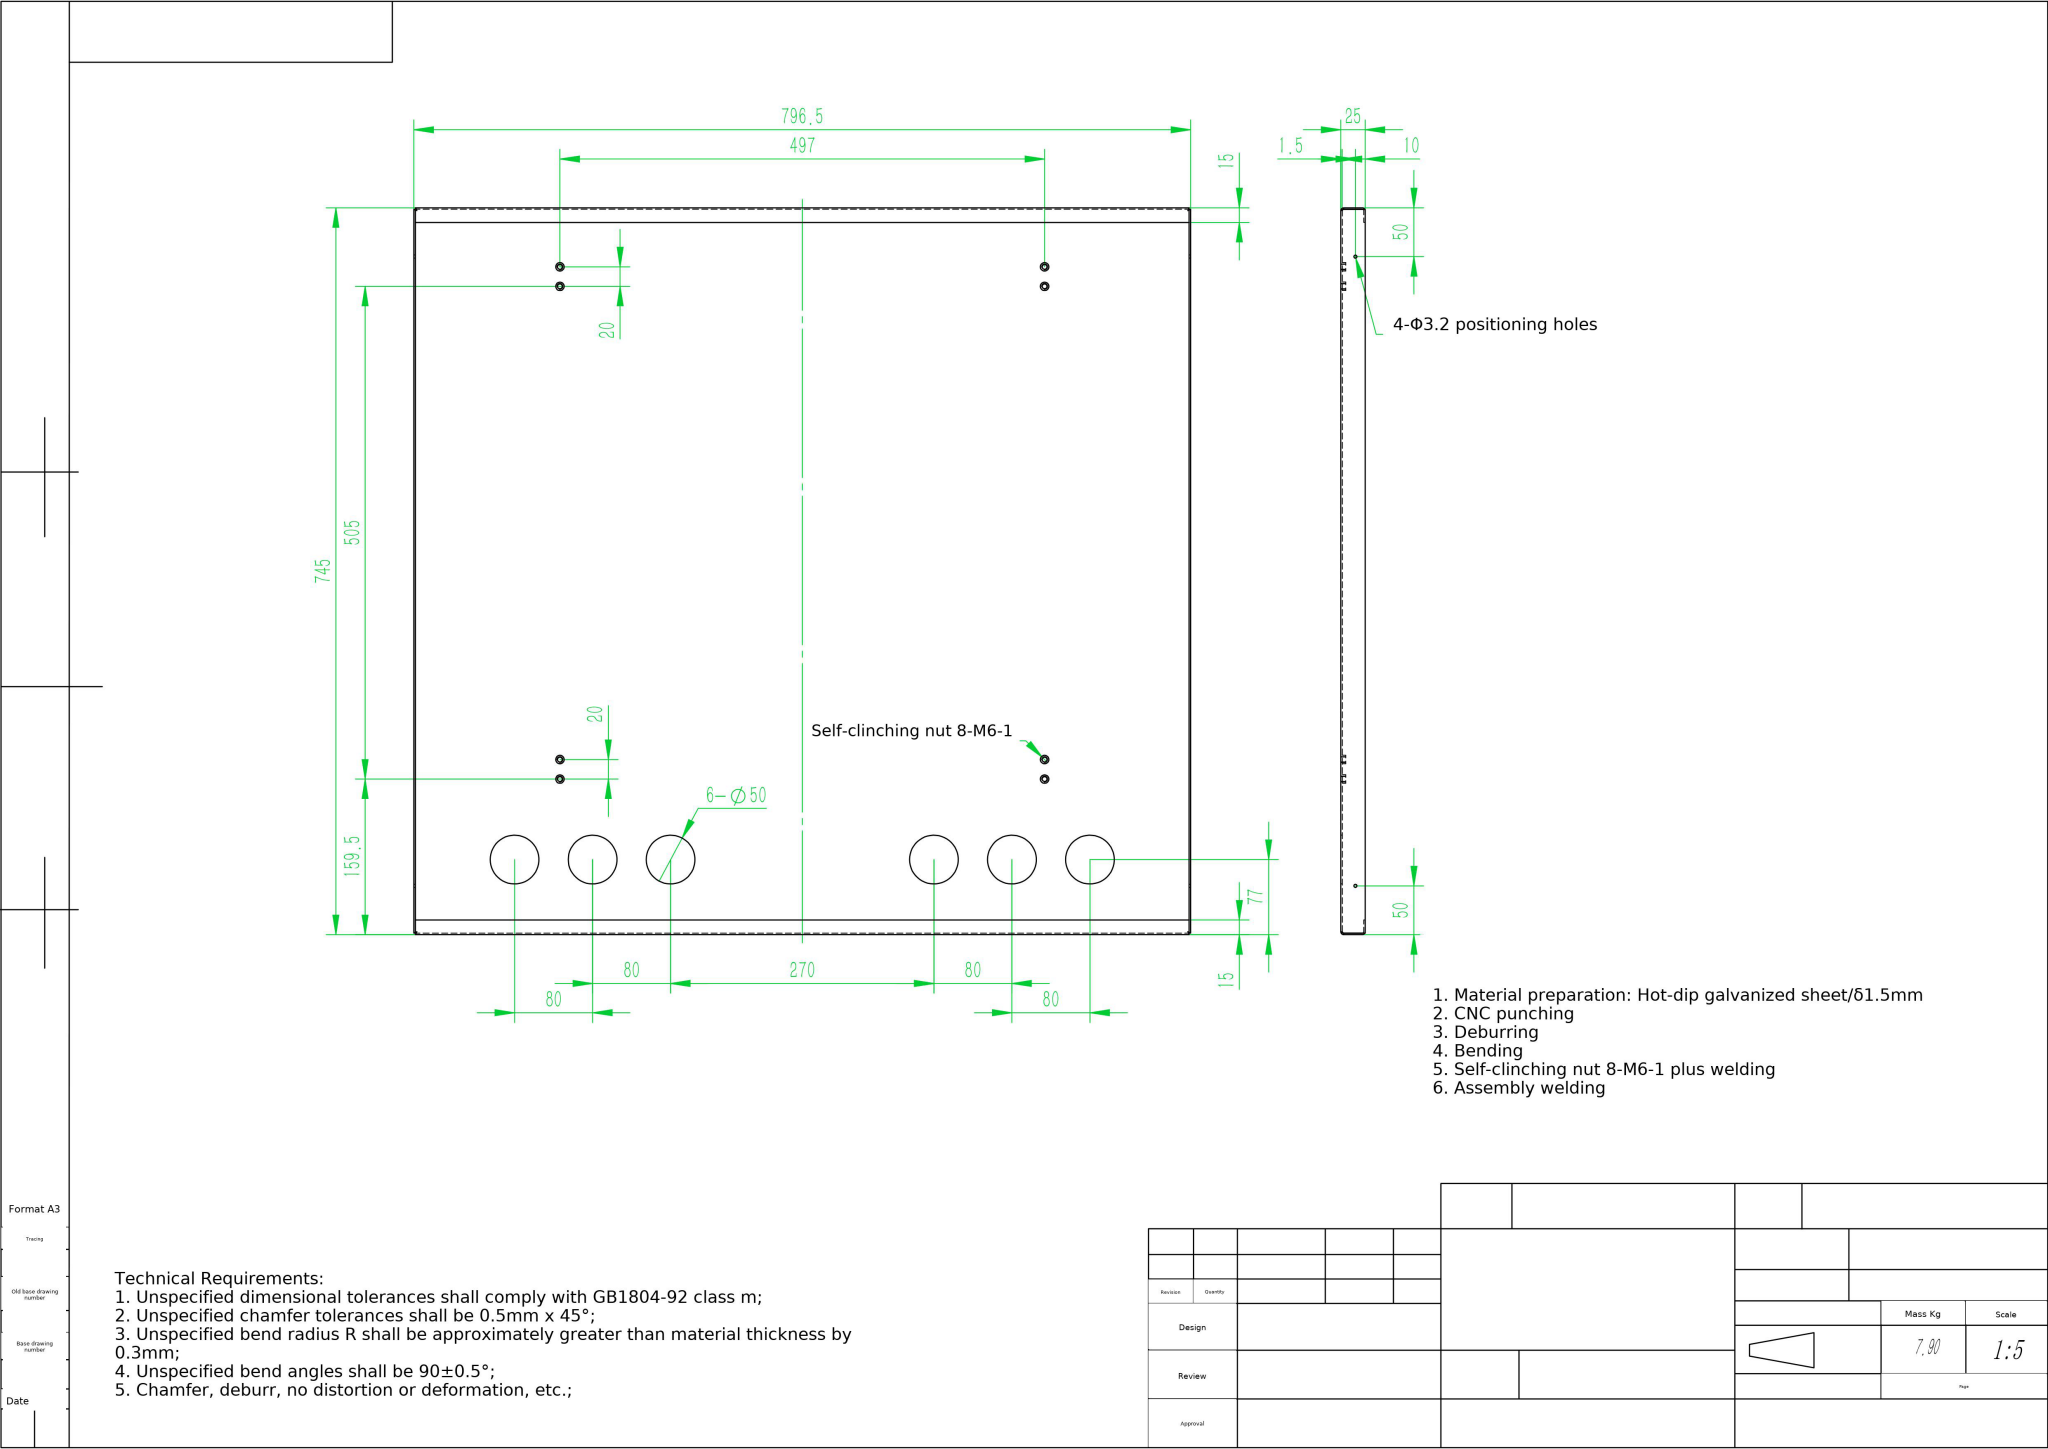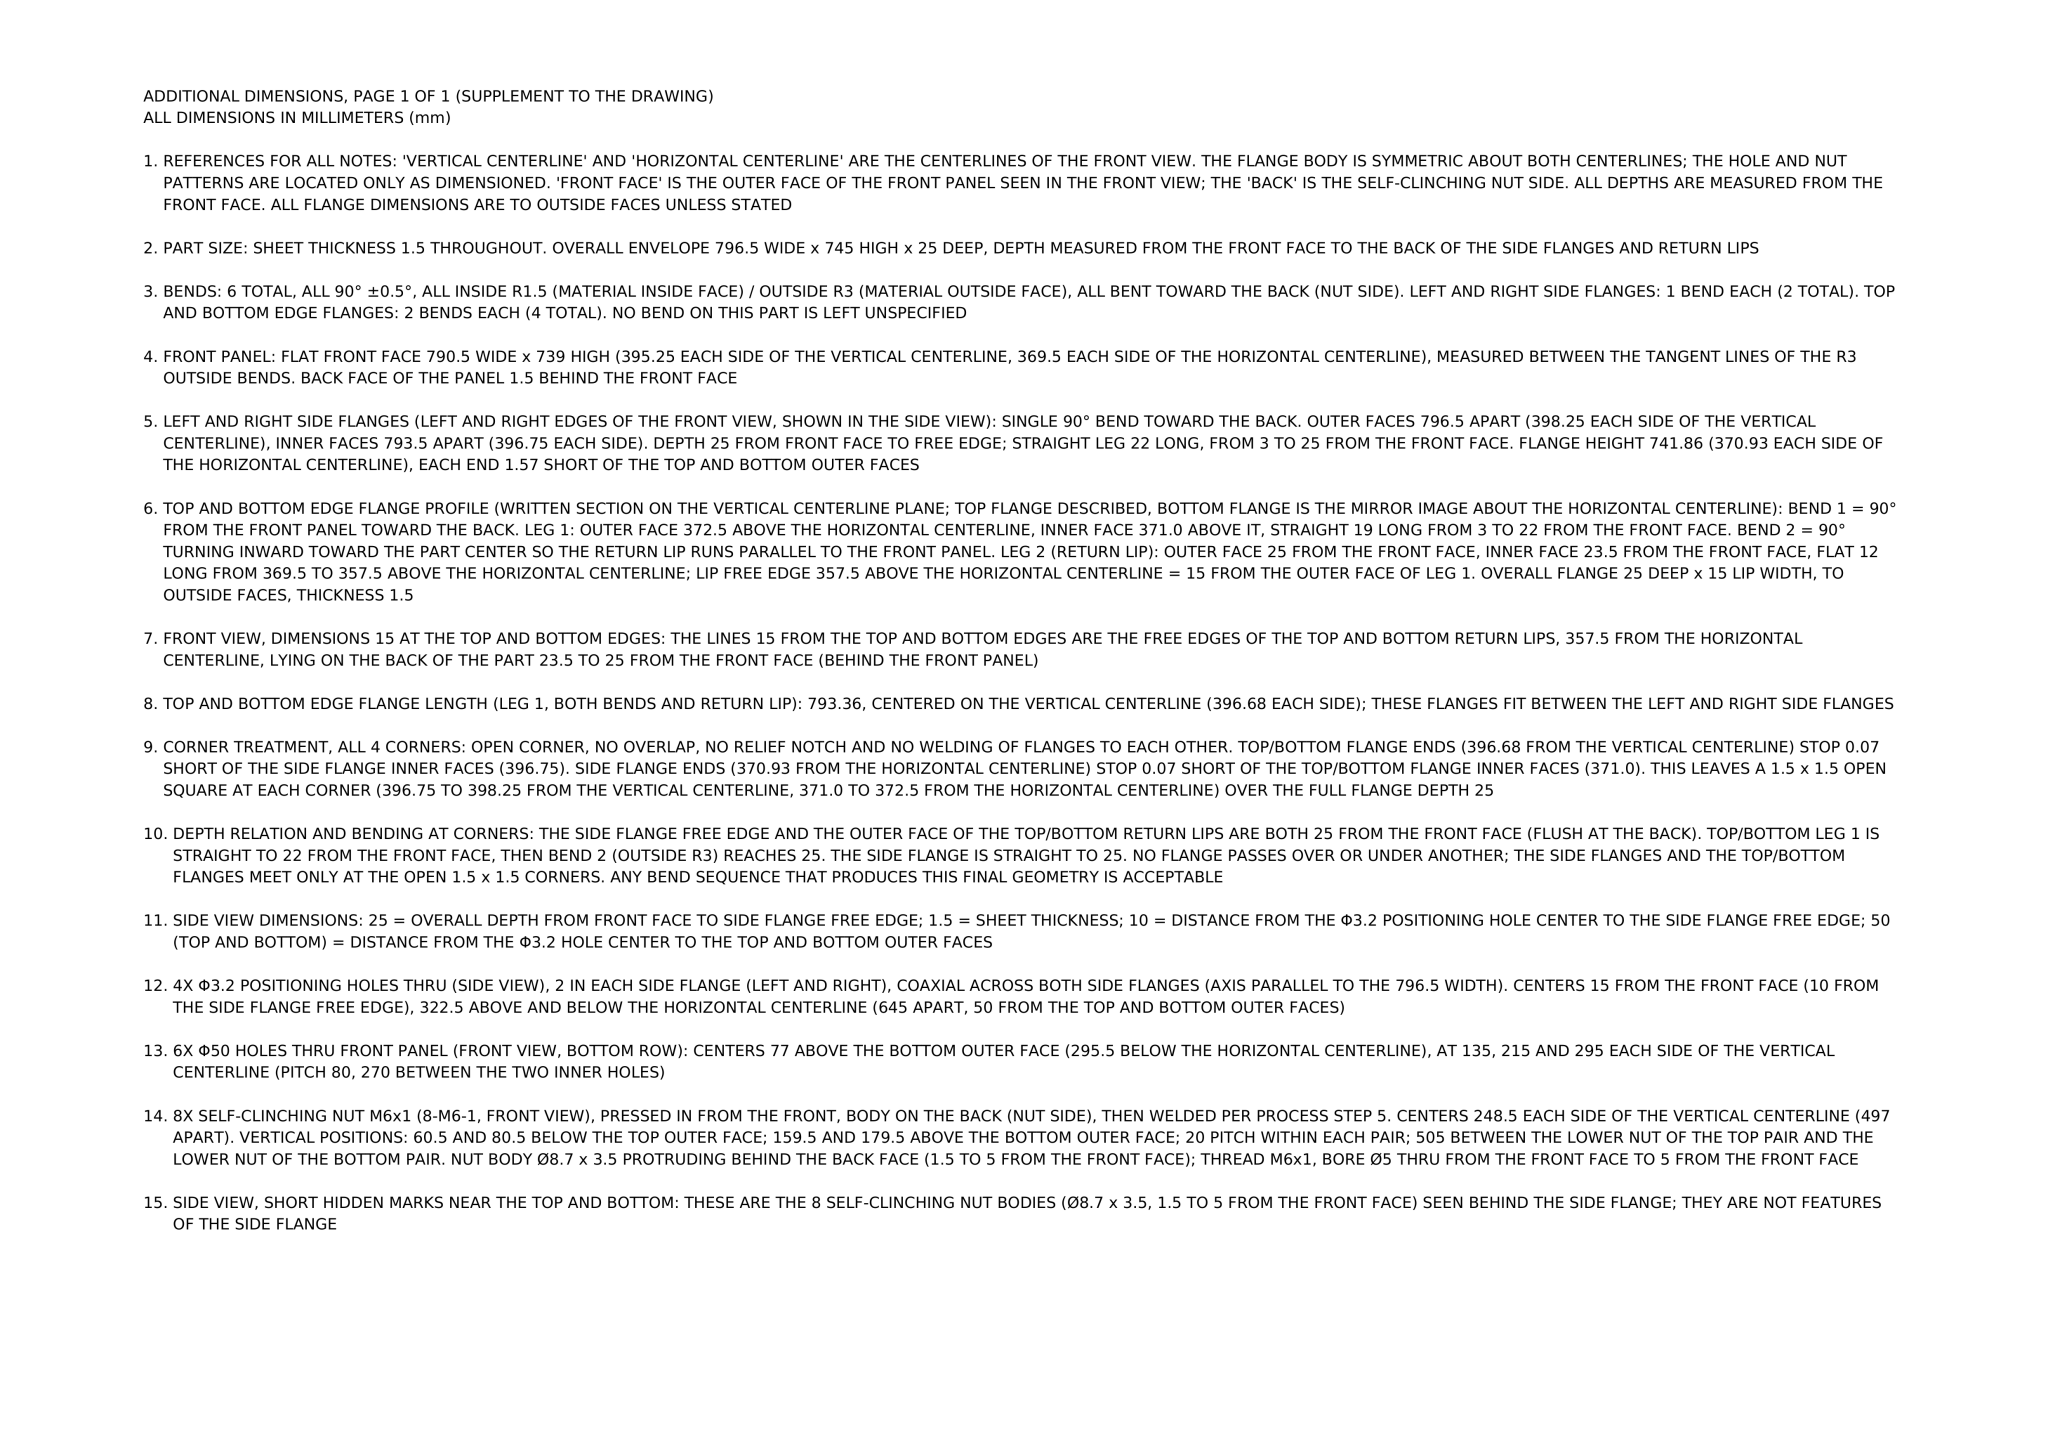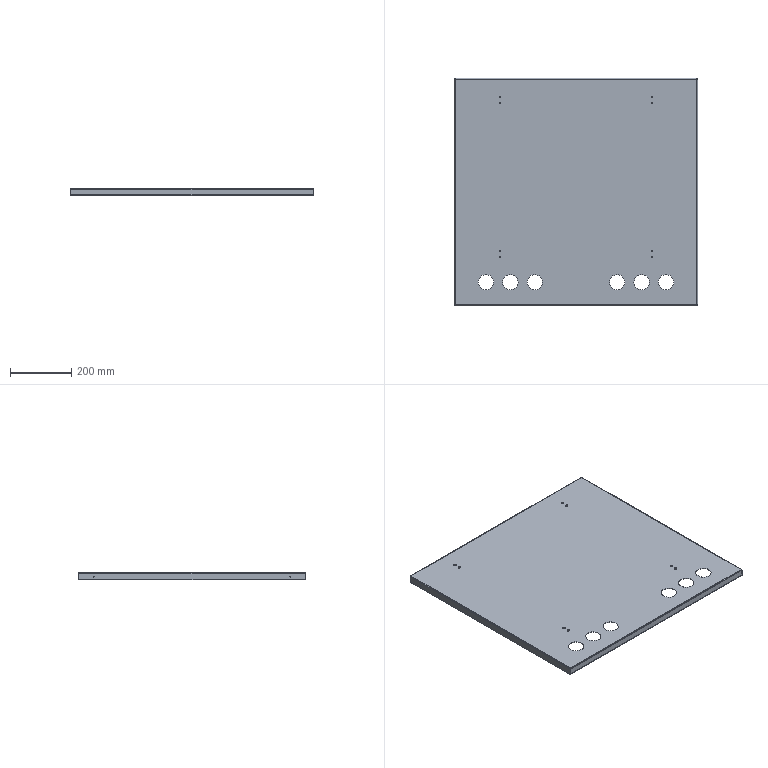Part | NX | mm | 1 solid | 114 faces | box 796.5 x 745 x 25 mm | volume 1006833 mm3 | cylinder 64 | plane 42 | spline 8 | commonest cylinder face diameters 5 x16 8.7 x16 50 x12 3.2 x8 6 x6 3 x6